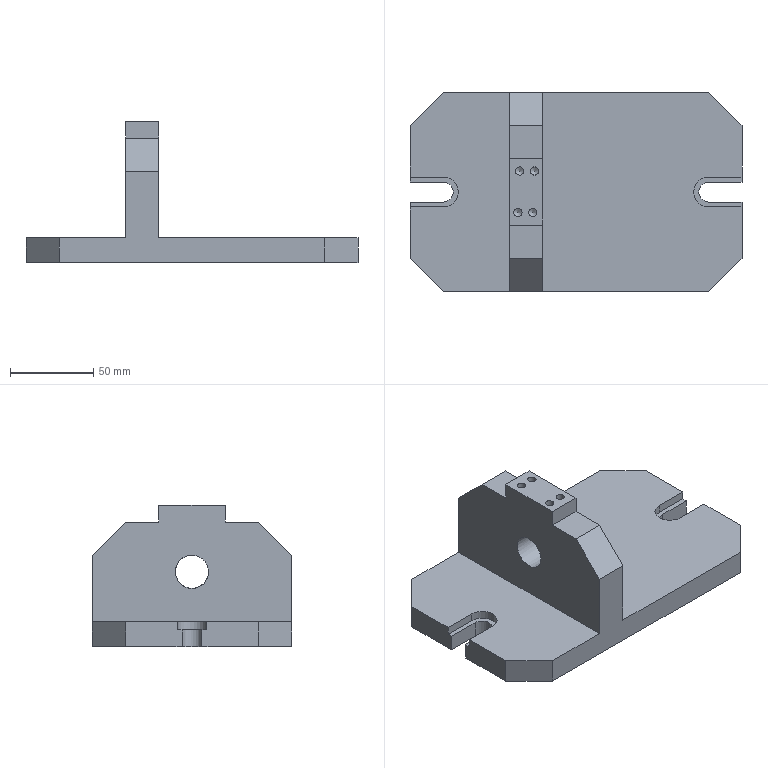Component | NX | FIXTURE_BODY | 1 solid | 59 faces | volume 471173 mm3 | plane 34 | cylinder 16 | cone 9 | commonest cylinder face diameters 6 x5 5 x4 12 x2 18 x2 20 x1 26 x1 8 x1